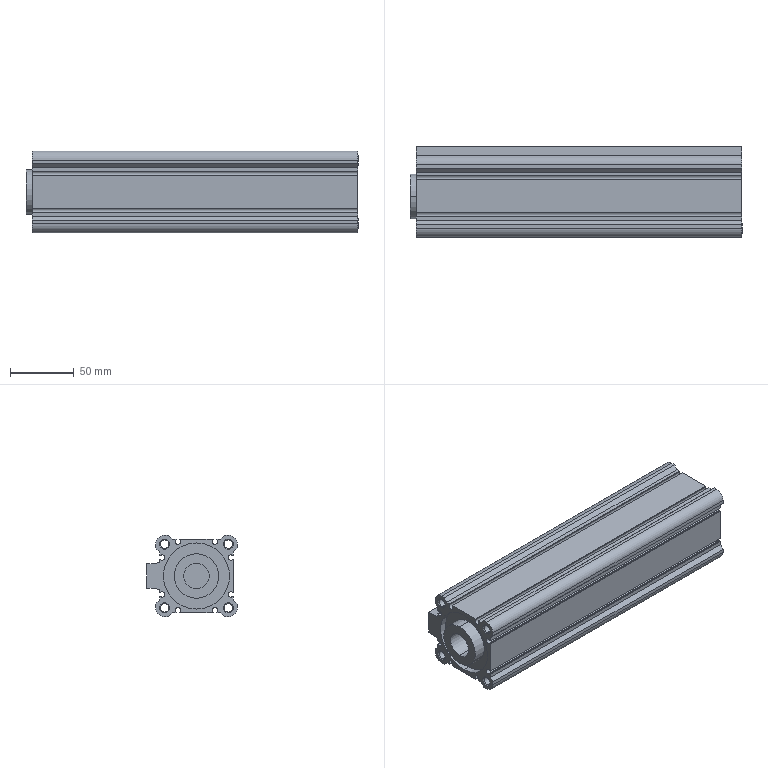Component | SolidWorks | CQ2A50-200DCZ(0_0_0)-1_CQ2A50-200DCZ(0_0_0)1-1 | 1 solid | 145 faces | volume 465943 mm3 | plane 65 | cylinder 60 | cone 20 | commonest cylinder face diameters 4.26 x18 6.647 x16 8 x8 52 x4 11.445 x4 14 x4 50 x2 20 x2